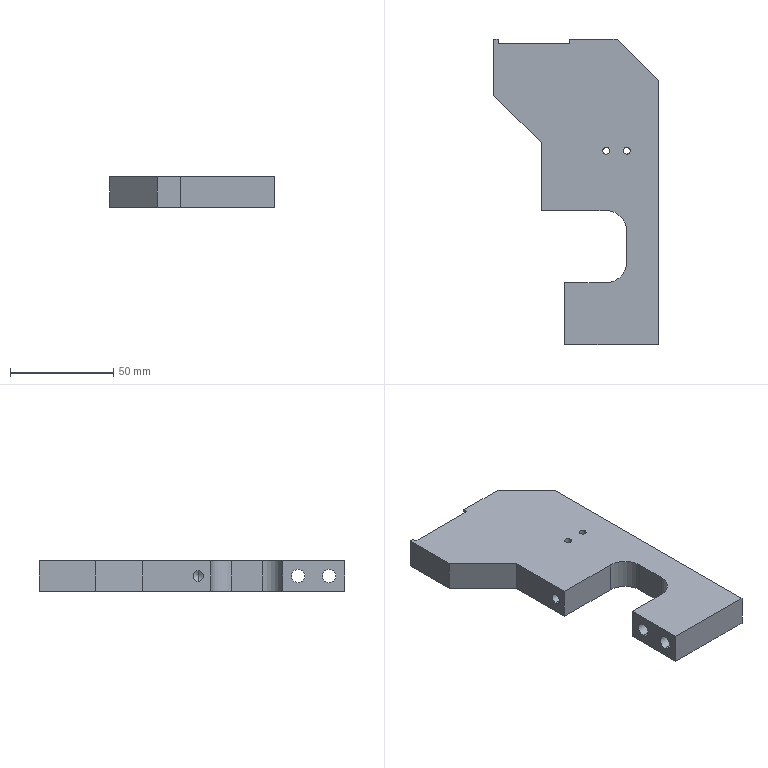Component | SolidWorks | WirePressingUnitSupportLeg-1 | 1 solid | 45 faces | volume 102839 mm3 | cylinder 20 | plane 19 | cone 6 | commonest cylinder face diameters 3.3 x4 4.2 x4 11 x4 6.5 x4 5 x2 20 x2